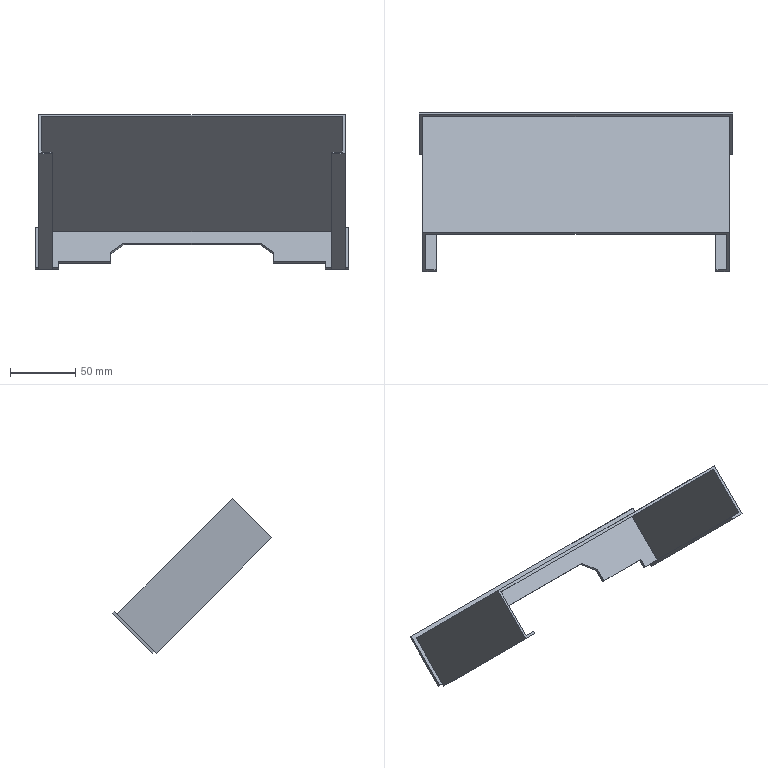Component | SolidWorks | Section4-1 | 2 solids | 30 faces | box 240 x 121.98 x 118.44 mm | volume 96218 mm3 | plane 30
build123d program:
from build123d import *

# Parameters (mm, degrees)
EXTRUDE_THIN1_DEPTH = 125
BOSS_EXTRUDE1_DEPTH = 2


with BuildPart() as part:
    # Sketch1 → Extrude-Thin1 (new body)
    with BuildSketch(Plane.XY):
        Polygon((2151.948, -29.605), (2141.948, -29.605), (2141.948, 12.895), (2375.948, 12.895), (2375.948, -29.605), (2365.948, -29.605), (2365.948, -27.605), (2373.948, -27.605), (2373.948, 10.895), (2143.948, 10.895), (2143.948, -27.605), (2151.948, -27.605), align=None)
    extrude(amount=EXTRUDE_THIN1_DEPTH)


with BuildPart() as body_2:
    # Sketch2 → Boss-Extrude1 (new body)
    with BuildSketch(Plane(origin=(0, 0, 0), x_dir=(-1, 0, 0), z_dir=(0, 0, -1))):
        Polygon((-2360.948, -27.605), (-2378.948, -27.605), (-2378.948, 15.895), (-2138.948, 15.895), (-2138.948, -27.605), (-2156.948, -27.605), (-2156.948, -21.105), (-2196.948, -21.105), (-2196.948, -11.105), (-2206.948, -1.105), (-2310.948, -1.105), (-2320.948, -11.105), (-2320.948, -21.105), (-2360.948, -21.105), align=None)
    extrude(amount=BOSS_EXTRUDE1_DEPTH)


solid = Compound([part.part, body_2.part])

# Placed as in the assembly
solid = solid.moved(Location((-2140.123, -346.52, 136.747), (45, 0, 0)))
STEP:
#1=COLOUR_RGB('',0.7922,0.8196,0.9333);
#2=FILL_AREA_STYLE_COLOUR('',#1);
#3=FILL_AREA_STYLE('',(#2));
#4=SURFACE_STYLE_FILL_AREA(#3);
#5=SURFACE_SIDE_STYLE('',(#4));
#6=SURFACE_STYLE_USAGE(.BOTH.,#5);
#7=PRESENTATION_STYLE_ASSIGNMENT((#6));
#8=CARTESIAN_POINT('',(8.694,-14.411,4.615));
#9=VERTEX_POINT('',#8);
#10=CARTESIAN_POINT('',(8.694,-14.23,4.796));
#11=VERTEX_POINT('',#10);
#12=CARTESIAN_POINT('',(8.694,-14.23,4.796));
#13=DIRECTION('',(-0.,0.7071,0.7071));
#14=VECTOR('',#13,39.37);
#15=LINE('',#12,#14);
#16=EDGE_CURVE('',#9,#11,#15,.T.);
#17=ORIENTED_EDGE('',*,*,#16,.T.);
#18=CARTESIAN_POINT('',(8.694,-14.174,4.741));
#19=VERTEX_POINT('',#18);
#20=CARTESIAN_POINT('',(8.694,-14.174,4.741));
#21=DIRECTION('',(0.,-0.7071,0.7071));
#22=VECTOR('',#21,39.37);
#23=LINE('',#20,#22);
#24=EDGE_CURVE('',#19,#11,#23,.T.);
#25=ORIENTED_EDGE('',*,*,#24,.F.);
#26=CARTESIAN_POINT('',(8.694,-14.355,4.56));
#27=VERTEX_POINT('',#26);
#28=CARTESIAN_POINT('',(8.694,-14.174,4.741));
#29=DIRECTION('',(-0.,0.7071,0.7071));
#30=VECTOR('',#29,39.37);
#31=LINE('',#28,#30);
#32=EDGE_CURVE('',#27,#19,#31,.T.);
#33=ORIENTED_EDGE('',*,*,#32,.F.);
#34=CARTESIAN_POINT('',(8.694,-14.355,4.56));
#35=DIRECTION('',(0.,-0.7071,0.7071));
#36=VECTOR('',#35,39.37);
#37=LINE('',#34,#36);
#38=EDGE_CURVE('',#27,#9,#37,.T.);
#39=ORIENTED_EDGE('',*,*,#38,.T.);
#40=EDGE_LOOP('',(#17,#25,#33,#39));
#41=FACE_OUTER_BOUND('',#40,.T.);
#42=CARTESIAN_POINT('',(8.694,-14.174,4.741));
#43=DIRECTION('',(1.,0.,-0.));
#44=DIRECTION('',(-0.,0.7071,-0.7071));
#45=AXIS2_PLACEMENT_3D('',#42,#43,#44);
#46=PLANE('',#45);
#47=ADVANCED_FACE('',(#41),#46,.F.);
#48=CARTESIAN_POINT('',(7.119,-14.23,4.796));
#49=VERTEX_POINT('',#48);
#50=CARTESIAN_POINT('',(7.119,-14.23,4.796));
#51=DIRECTION('',(-1.,-0.,0.));
#52=VECTOR('',#51,39.37);
#53=LINE('',#50,#52);
#54=EDGE_CURVE('',#11,#49,#53,.T.);
#55=ORIENTED_EDGE('',*,*,#54,.T.);
#56=CARTESIAN_POINT('',(7.119,-14.174,4.741));
#57=VERTEX_POINT('',#56);
#58=CARTESIAN_POINT('',(7.119,-14.174,4.741));
#59=DIRECTION('',(0.,-0.7071,0.7071));
#60=VECTOR('',#59,39.37);
#61=LINE('',#58,#60);
#62=EDGE_CURVE('',#57,#49,#61,.T.);
#63=ORIENTED_EDGE('',*,*,#62,.F.);
#64=CARTESIAN_POINT('',(7.119,-14.174,4.741));
#65=DIRECTION('',(-1.,-0.,0.));
#66=VECTOR('',#65,39.37);
#67=LINE('',#64,#66);
#68=EDGE_CURVE('',#19,#57,#67,.T.);
#69=ORIENTED_EDGE('',*,*,#68,.F.);
#70=ORIENTED_EDGE('',*,*,#24,.T.);
#71=EDGE_LOOP('',(#55,#63,#69,#70));
#72=FACE_OUTER_BOUND('',#71,.T.);
#73=CARTESIAN_POINT('',(7.119,-14.174,4.741));
#74=DIRECTION('',(0.,0.7071,0.7071));
#75=DIRECTION('',(-1.,-0.,0.));
#76=AXIS2_PLACEMENT_3D('',#73,#74,#75);
#77=PLANE('',#76);
#78=ADVANCED_FACE('',(#72),#77,.F.);
#79=CARTESIAN_POINT('',(7.119,-13.952,5.075));
#80=VERTEX_POINT('',#79);
#81=CARTESIAN_POINT('',(7.119,-13.952,5.075));
#82=DIRECTION('',(0.,0.7071,0.7071));
#83=VECTOR('',#82,39.37);
#84=LINE('',#81,#83);
#85=EDGE_CURVE('',#49,#80,#84,.T.);
#86=ORIENTED_EDGE('',*,*,#85,.T.);
#87=CARTESIAN_POINT('',(7.119,-13.896,5.019));
#88=VERTEX_POINT('',#87);
#89=CARTESIAN_POINT('',(7.119,-13.896,5.019));
#90=DIRECTION('',(0.,-0.7071,0.7071));
#91=VECTOR('',#90,39.37);
#92=LINE('',#89,#91);
#93=EDGE_CURVE('',#88,#80,#92,.T.);
#94=ORIENTED_EDGE('',*,*,#93,.F.);
#95=CARTESIAN_POINT('',(7.119,-13.896,5.019));
#96=DIRECTION('',(0.,0.7071,0.7071));
#97=VECTOR('',#96,39.37);
#98=LINE('',#95,#97);
#99=EDGE_CURVE('',#57,#88,#98,.T.);
#100=ORIENTED_EDGE('',*,*,#99,.F.);
#101=ORIENTED_EDGE('',*,*,#62,.T.);
#102=EDGE_LOOP('',(#86,#94,#100,#101));
#103=FACE_OUTER_BOUND('',#102,.T.);
#104=CARTESIAN_POINT('',(7.119,-13.896,5.019));
#105=DIRECTION('',(1.,-0.,-0.));
#106=DIRECTION('',(0.,0.7071,0.7071));
#107=AXIS2_PLACEMENT_3D('',#104,#105,#106);
#108=PLANE('',#107);
#109=ADVANCED_FACE('',(#103),#108,.F.);
#110=CARTESIAN_POINT('',(6.725,-13.673,5.353));
#111=VERTEX_POINT('',#110);
#112=CARTESIAN_POINT('',(6.725,-13.673,5.353));
#113=DIRECTION('',(-0.7071,0.5,0.5));
#114=VECTOR('',#113,39.37);
#115=LINE('',#112,#114);
#116=EDGE_CURVE('',#80,#111,#115,.T.);
#117=ORIENTED_EDGE('',*,*,#116,.T.);
#118=CARTESIAN_POINT('',(6.725,-13.618,5.297));
#119=VERTEX_POINT('',#118);
#120=CARTESIAN_POINT('',(6.725,-13.618,5.297));
#121=DIRECTION('',(0.,-0.7071,0.7071));
#122=VECTOR('',#121,39.37);
#123=LINE('',#120,#122);
#124=EDGE_CURVE('',#119,#111,#123,.T.);
#125=ORIENTED_EDGE('',*,*,#124,.F.);
#126=CARTESIAN_POINT('',(6.725,-13.618,5.297));
#127=DIRECTION('',(-0.7071,0.5,0.5));
#128=VECTOR('',#127,39.37);
#129=LINE('',#126,#128);
#130=EDGE_CURVE('',#88,#119,#129,.T.);
#131=ORIENTED_EDGE('',*,*,#130,.F.);
#132=ORIENTED_EDGE('',*,*,#93,.T.);
#133=EDGE_LOOP('',(#117,#125,#131,#132));
#134=FACE_OUTER_BOUND('',#133,.T.);
#135=CARTESIAN_POINT('',(6.725,-13.618,5.297));
#136=DIRECTION('',(0.7071,0.5,0.5));
#137=DIRECTION('',(-0.7071,0.5,0.5));
#138=AXIS2_PLACEMENT_3D('',#135,#136,#137);
#139=PLANE('',#138);
#140=ADVANCED_FACE('',(#134),#139,.F.);
#141=CARTESIAN_POINT('',(2.631,-13.673,5.353));
#142=VERTEX_POINT('',#141);
#143=CARTESIAN_POINT('',(2.631,-13.673,5.353));
#144=DIRECTION('',(-1.,-0.,0.));
#145=VECTOR('',#144,39.37);
#146=LINE('',#143,#145);
#147=EDGE_CURVE('',#111,#142,#146,.T.);
#148=ORIENTED_EDGE('',*,*,#147,.T.);
#149=CARTESIAN_POINT('',(2.631,-13.618,5.297));
#150=VERTEX_POINT('',#149);
#151=CARTESIAN_POINT('',(2.631,-13.618,5.297));
#152=DIRECTION('',(0.,-0.7071,0.7071));
#153=VECTOR('',#152,39.37);
#154=LINE('',#151,#153);
#155=EDGE_CURVE('',#150,#142,#154,.T.);
#156=ORIENTED_EDGE('',*,*,#155,.F.);
#157=CARTESIAN_POINT('',(2.631,-13.618,5.297));
#158=DIRECTION('',(-1.,-0.,0.));
#159=VECTOR('',#158,39.37);
#160=LINE('',#157,#159);
#161=EDGE_CURVE('',#119,#150,#160,.T.);
#162=ORIENTED_EDGE('',*,*,#161,.F.);
#163=ORIENTED_EDGE('',*,*,#124,.T.);
#164=EDGE_LOOP('',(#148,#156,#162,#163));
#165=FACE_OUTER_BOUND('',#164,.T.);
#166=CARTESIAN_POINT('',(2.631,-13.618,5.297));
#167=DIRECTION('',(0.,0.7071,0.7071));
#168=DIRECTION('',(-1.,-0.,0.));
#169=AXIS2_PLACEMENT_3D('',#166,#167,#168);
#170=PLANE('',#169);
#171=ADVANCED_FACE('',(#165),#170,.F.);
#172=CARTESIAN_POINT('',(2.237,-13.952,5.075));
#173=VERTEX_POINT('',#172);
#174=CARTESIAN_POINT('',(2.237,-13.952,5.075));
#175=DIRECTION('',(-0.7071,-0.5,-0.5));
#176=VECTOR('',#175,39.37);
#177=LINE('',#174,#176);
#178=EDGE_CURVE('',#142,#173,#177,.T.);
#179=ORIENTED_EDGE('',*,*,#178,.T.);
#180=CARTESIAN_POINT('',(2.237,-13.896,5.019));
#181=VERTEX_POINT('',#180);
#182=CARTESIAN_POINT('',(2.237,-13.896,5.019));
#183=DIRECTION('',(0.,-0.7071,0.7071));
#184=VECTOR('',#183,39.37);
#185=LINE('',#182,#184);
#186=EDGE_CURVE('',#181,#173,#185,.T.);
#187=ORIENTED_EDGE('',*,*,#186,.F.);
#188=CARTESIAN_POINT('',(2.237,-13.896,5.019));
#189=DIRECTION('',(-0.7071,-0.5,-0.5));
#190=VECTOR('',#189,39.37);
#191=LINE('',#188,#190);
#192=EDGE_CURVE('',#150,#181,#191,.T.);
#193=ORIENTED_EDGE('',*,*,#192,.F.);
#194=ORIENTED_EDGE('',*,*,#155,.T.);
#195=EDGE_LOOP('',(#179,#187,#193,#194));
#196=FACE_OUTER_BOUND('',#195,.T.);
#197=CARTESIAN_POINT('',(2.237,-13.896,5.019));
#198=DIRECTION('',(-0.7071,0.5,0.5));
#199=DIRECTION('',(-0.7071,-0.5,-0.5));
#200=AXIS2_PLACEMENT_3D('',#197,#198,#199);
#201=PLANE('',#200);
#202=ADVANCED_FACE('',(#196),#201,.F.);
#203=CARTESIAN_POINT('',(2.237,-14.23,4.796));
#204=VERTEX_POINT('',#203);
#205=CARTESIAN_POINT('',(2.237,-14.23,4.796));
#206=DIRECTION('',(-0.,-0.7071,-0.7071));
#207=VECTOR('',#206,39.37);
#208=LINE('',#205,#207);
#209=EDGE_CURVE('',#173,#204,#208,.T.);
#210=ORIENTED_EDGE('',*,*,#209,.T.);
#211=CARTESIAN_POINT('',(2.237,-14.174,4.741));
#212=VERTEX_POINT('',#211);
#213=CARTESIAN_POINT('',(2.237,-14.174,4.741));
#214=DIRECTION('',(0.,-0.7071,0.7071));
#215=VECTOR('',#214,39.37);
#216=LINE('',#213,#215);
#217=EDGE_CURVE('',#212,#204,#216,.T.);
#218=ORIENTED_EDGE('',*,*,#217,.F.);
#219=CARTESIAN_POINT('',(2.237,-14.174,4.741));
#220=DIRECTION('',(-0.,-0.7071,-0.7071));
#221=VECTOR('',#220,39.37);
#222=LINE('',#219,#221);
#223=EDGE_CURVE('',#181,#212,#222,.T.);
#224=ORIENTED_EDGE('',*,*,#223,.F.);
#225=ORIENTED_EDGE('',*,*,#186,.T.);
#226=EDGE_LOOP('',(#210,#218,#224,#225));
#227=FACE_OUTER_BOUND('',#226,.T.);
#228=CARTESIAN_POINT('',(2.237,-14.174,4.741));
#229=DIRECTION('',(-1.,0.,0.));
#230=DIRECTION('',(-0.,-0.7071,-0.7071));
#231=AXIS2_PLACEMENT_3D('',#228,#229,#230);
#232=PLANE('',#231);
#233=ADVANCED_FACE('',(#227),#232,.F.);
#234=CARTESIAN_POINT('',(0.6624,-14.23,4.796));
#235=VERTEX_POINT('',#234);
#236=CARTESIAN_POINT('',(0.6624,-14.23,4.796));
#237=DIRECTION('',(-1.,-0.,0.));
#238=VECTOR('',#237,39.37);
#239=LINE('',#236,#238);
#240=EDGE_CURVE('',#204,#235,#239,.T.);
#241=ORIENTED_EDGE('',*,*,#240,.T.);
#242=CARTESIAN_POINT('',(0.6624,-14.174,4.741));
#243=VERTEX_POINT('',#242);
#244=CARTESIAN_POINT('',(0.6624,-14.174,4.741));
#245=DIRECTION('',(0.,-0.7071,0.7071));
#246=VECTOR('',#245,39.37);
#247=LINE('',#244,#246);
#248=EDGE_CURVE('',#243,#235,#247,.T.);
#249=ORIENTED_EDGE('',*,*,#248,.F.);
#250=CARTESIAN_POINT('',(0.6624,-14.174,4.741));
#251=DIRECTION('',(-1.,-0.,0.));
#252=VECTOR('',#251,39.37);
#253=LINE('',#250,#252);
#254=EDGE_CURVE('',#212,#243,#253,.T.);
#255=ORIENTED_EDGE('',*,*,#254,.F.);
#256=ORIENTED_EDGE('',*,*,#217,.T.);
#257=EDGE_LOOP('',(#241,#249,#255,#256));
#258=FACE_OUTER_BOUND('',#257,.T.);
#259=CARTESIAN_POINT('',(0.6624,-14.174,4.741));
#260=DIRECTION('',(0.,0.7071,0.7071));
#261=DIRECTION('',(-1.,-0.,0.));
#262=AXIS2_PLACEMENT_3D('',#259,#260,#261);
#263=PLANE('',#262);
#264=ADVANCED_FACE('',(#258),#263,.F.);
#265=CARTESIAN_POINT('',(0.6624,-14.411,4.615));
#266=VERTEX_POINT('',#265);
#267=CARTESIAN_POINT('',(0.6624,-14.411,4.615));
#268=DIRECTION('',(0.,-0.7071,-0.7071));
#269=VECTOR('',#268,39.37);
#270=LINE('',#267,#269);
#271=EDGE_CURVE('',#235,#266,#270,.T.);
#272=ORIENTED_EDGE('',*,*,#271,.T.);
#273=CARTESIAN_POINT('',(0.6624,-14.355,4.56));
#274=VERTEX_POINT('',#273);
#275=CARTESIAN_POINT('',(0.6624,-14.355,4.56));
#276=DIRECTION('',(0.,-0.7071,0.7071));
#277=VECTOR('',#276,39.37);
#278=LINE('',#275,#277);
#279=EDGE_CURVE('',#274,#266,#278,.T.);
#280=ORIENTED_EDGE('',*,*,#279,.F.);
#281=CARTESIAN_POINT('',(0.6624,-14.355,4.56));
#282=DIRECTION('',(0.,-0.7071,-0.7071));
#283=VECTOR('',#282,39.37);
#284=LINE('',#281,#283);
#285=EDGE_CURVE('',#243,#274,#284,.T.);
#286=ORIENTED_EDGE('',*,*,#285,.F.);
#287=ORIENTED_EDGE('',*,*,#248,.T.);
#288=EDGE_LOOP('',(#272,#280,#286,#287));
#289=FACE_OUTER_BOUND('',#288,.T.);
#290=CARTESIAN_POINT('',(0.6624,-14.355,4.56));
#291=DIRECTION('',(-1.,-0.,0.));
#292=DIRECTION('',(0.,-0.7071,0.7071));
#293=AXIS2_PLACEMENT_3D('',#290,#291,#292);
#294=PLANE('',#293);
#295=ADVANCED_FACE('',(#289),#294,.F.);
#296=CARTESIAN_POINT('',(-0.04628,-14.411,4.615));
#297=VERTEX_POINT('',#296);
#298=CARTESIAN_POINT('',(-0.04628,-14.411,4.615));
#299=DIRECTION('',(-1.,-0.,0.));
#300=VECTOR('',#299,39.37);
#301=LINE('',#298,#300);
#302=EDGE_CURVE('',#266,#297,#301,.T.);
#303=ORIENTED_EDGE('',*,*,#302,.T.);
#304=CARTESIAN_POINT('',(-0.04628,-14.355,4.56));
#305=VERTEX_POINT('',#304);
#306=CARTESIAN_POINT('',(-0.04628,-14.355,4.56));
#307=DIRECTION('',(0.,-0.7071,0.7071));
#308=VECTOR('',#307,39.37);
#309=LINE('',#306,#308);
#310=EDGE_CURVE('',#305,#297,#309,.T.);
#311=ORIENTED_EDGE('',*,*,#310,.F.);
#312=CARTESIAN_POINT('',(-0.04628,-14.355,4.56));
#313=DIRECTION('',(-1.,-0.,0.));
#314=VECTOR('',#313,39.37);
#315=LINE('',#312,#314);
#316=EDGE_CURVE('',#274,#305,#315,.T.);
#317=ORIENTED_EDGE('',*,*,#316,.F.);
#318=ORIENTED_EDGE('',*,*,#279,.T.);
#319=EDGE_LOOP('',(#303,#311,#317,#318));
#320=FACE_OUTER_BOUND('',#319,.T.);
#321=CARTESIAN_POINT('',(-0.04628,-14.355,4.56));
#322=DIRECTION('',(-0.,0.7071,0.7071));
#323=DIRECTION('',(0.,-0.7071,0.7071));
#324=AXIS2_PLACEMENT_3D('',#321,#322,#323);
#325=PLANE('',#324);
#326=ADVANCED_FACE('',(#320),#325,.F.);
#327=CARTESIAN_POINT('',(-0.04628,-13.2,5.826));
#328=VERTEX_POINT('',#327);
#329=CARTESIAN_POINT('',(-0.04628,-13.2,5.826));
#330=DIRECTION('',(-0.,0.7071,0.7071));
#331=VECTOR('',#330,39.37);
#332=LINE('',#329,#331);
#333=EDGE_CURVE('',#297,#328,#332,.T.);
#334=ORIENTED_EDGE('',*,*,#333,.T.);
#335=CARTESIAN_POINT('',(-0.04628,-13.144,5.771));
#336=VERTEX_POINT('',#335);
#337=CARTESIAN_POINT('',(-0.04628,-13.144,5.771));
#338=DIRECTION('',(0.,-0.7071,0.7071));
#339=VECTOR('',#338,39.37);
#340=LINE('',#337,#339);
#341=EDGE_CURVE('',#336,#328,#340,.T.);
#342=ORIENTED_EDGE('',*,*,#341,.F.);
#343=CARTESIAN_POINT('',(-0.04628,-13.144,5.771));
#344=DIRECTION('',(-0.,0.7071,0.7071));
#345=VECTOR('',#344,39.37);
#346=LINE('',#343,#345);
#347=EDGE_CURVE('',#305,#336,#346,.T.);
#348=ORIENTED_EDGE('',*,*,#347,.F.);
#349=ORIENTED_EDGE('',*,*,#310,.T.);
#350=EDGE_LOOP('',(#334,#342,#348,#349));
#351=FACE_OUTER_BOUND('',#350,.T.);
#352=CARTESIAN_POINT('',(-0.04628,-13.144,5.771));
#353=DIRECTION('',(1.,0.,-0.));
#354=DIRECTION('',(-0.,0.7071,-0.7071));
#355=AXIS2_PLACEMENT_3D('',#352,#353,#354);
#356=PLANE('',#355);
#357=ADVANCED_FACE('',(#351),#356,.F.);
#358=CARTESIAN_POINT('',(9.403,-13.2,5.826));
#359=VERTEX_POINT('',#358);
#360=CARTESIAN_POINT('',(9.403,-13.2,5.826));
#361=DIRECTION('',(1.,0.,-0.));
#362=VECTOR('',#361,39.37);
#363=LINE('',#360,#362);
#364=EDGE_CURVE('',#328,#359,#363,.T.);
#365=ORIENTED_EDGE('',*,*,#364,.T.);
#366=CARTESIAN_POINT('',(9.403,-13.144,5.771));
#367=VERTEX_POINT('',#366);
#368=CARTESIAN_POINT('',(9.403,-13.144,5.771));
#369=DIRECTION('',(0.,-0.7071,0.7071));
#370=VECTOR('',#369,39.37);
#371=LINE('',#368,#370);
#372=EDGE_CURVE('',#367,#359,#371,.T.);
#373=ORIENTED_EDGE('',*,*,#372,.F.);
#374=CARTESIAN_POINT('',(9.403,-13.144,5.771));
#375=DIRECTION('',(1.,0.,-0.));
#376=VECTOR('',#375,39.37);
#377=LINE('',#374,#376);
#378=EDGE_CURVE('',#336,#367,#377,.T.);
#379=ORIENTED_EDGE('',*,*,#378,.F.);
#380=ORIENTED_EDGE('',*,*,#341,.T.);
#381=EDGE_LOOP('',(#365,#373,#379,#380));
#382=FACE_OUTER_BOUND('',#381,.T.);
#383=CARTESIAN_POINT('',(9.403,-13.144,5.771));
#384=DIRECTION('',(0.,-0.7071,-0.7071));
#385=DIRECTION('',(-0.,0.7071,-0.7071));
#386=AXIS2_PLACEMENT_3D('',#383,#384,#385);
#387=PLANE('',#386);
#388=ADVANCED_FACE('',(#382),#387,.F.);
#389=CARTESIAN_POINT('',(9.403,-14.411,4.615));
#390=VERTEX_POINT('',#389);
#391=CARTESIAN_POINT('',(9.403,-14.411,4.615));
#392=DIRECTION('',(0.,-0.7071,-0.7071));
#393=VECTOR('',#392,39.37);
#394=LINE('',#391,#393);
#395=EDGE_CURVE('',#359,#390,#394,.T.);
#396=ORIENTED_EDGE('',*,*,#395,.T.);
#397=CARTESIAN_POINT('',(9.403,-14.355,4.56));
#398=VERTEX_POINT('',#397);
#399=CARTESIAN_POINT('',(9.403,-14.355,4.56));
#400=DIRECTION('',(0.,-0.7071,0.7071));
#401=VECTOR('',#400,39.37);
#402=LINE('',#399,#401);
#403=EDGE_CURVE('',#398,#390,#402,.T.);
#404=ORIENTED_EDGE('',*,*,#403,.F.);
#405=CARTESIAN_POINT('',(9.403,-14.355,4.56));
#406=DIRECTION('',(0.,-0.7071,-0.7071));
#407=VECTOR('',#406,39.37);
#408=LINE('',#405,#407);
#409=EDGE_CURVE('',#367,#398,#408,.T.);
#410=ORIENTED_EDGE('',*,*,#409,.F.);
#411=ORIENTED_EDGE('',*,*,#372,.T.);
#412=EDGE_LOOP('',(#396,#404,#410,#411));
#413=FACE_OUTER_BOUND('',#412,.T.);
#414=CARTESIAN_POINT('',(9.403,-14.355,4.56));
#415=DIRECTION('',(-1.,-0.,0.));
#416=DIRECTION('',(0.,-0.7071,0.7071));
#417=AXIS2_PLACEMENT_3D('',#414,#415,#416);
#418=PLANE('',#417);
#419=ADVANCED_FACE('',(#413),#418,.F.);
#420=CARTESIAN_POINT('',(8.694,-14.411,4.615));
#421=DIRECTION('',(-1.,-0.,0.));
#422=VECTOR('',#421,39.37);
#423=LINE('',#420,#422);
#424=EDGE_CURVE('',#390,#9,#423,.T.);
#425=ORIENTED_EDGE('',*,*,#424,.T.);
#426=ORIENTED_EDGE('',*,*,#38,.F.);
#427=CARTESIAN_POINT('',(8.694,-14.355,4.56));
#428=DIRECTION('',(-1.,-0.,0.));
#429=VECTOR('',#428,39.37);
#430=LINE('',#427,#429);
#431=EDGE_CURVE('',#398,#27,#430,.T.);
#432=ORIENTED_EDGE('',*,*,#431,.F.);
#433=ORIENTED_EDGE('',*,*,#403,.T.);
#434=EDGE_LOOP('',(#425,#426,#432,#433));
#435=FACE_OUTER_BOUND('',#434,.T.);
#436=CARTESIAN_POINT('',(8.694,-14.355,4.56));
#437=DIRECTION('',(-0.,0.7071,0.7071));
#438=DIRECTION('',(0.,-0.7071,0.7071));
#439=AXIS2_PLACEMENT_3D('',#436,#437,#438);
#440=PLANE('',#439);
#441=ADVANCED_FACE('',(#435),#440,.F.);
#442=ORIENTED_EDGE('',*,*,#32,.T.);
#443=ORIENTED_EDGE('',*,*,#68,.T.);
#444=ORIENTED_EDGE('',*,*,#99,.T.);
#445=ORIENTED_EDGE('',*,*,#130,.T.);
#446=ORIENTED_EDGE('',*,*,#161,.T.);
#447=ORIENTED_EDGE('',*,*,#192,.T.);
#448=ORIENTED_EDGE('',*,*,#223,.T.);
#449=ORIENTED_EDGE('',*,*,#254,.T.);
#450=ORIENTED_EDGE('',*,*,#285,.T.);
#451=ORIENTED_EDGE('',*,*,#316,.T.);
#452=ORIENTED_EDGE('',*,*,#347,.T.);
#453=ORIENTED_EDGE('',*,*,#378,.T.);
#454=ORIENTED_EDGE('',*,*,#409,.T.);
#455=ORIENTED_EDGE('',*,*,#431,.T.);
#456=EDGE_LOOP('',(#442,#443,#444,#445,#446,#447,#448,#449,#450,#451,#452,#453,#454,#455));
#457=FACE_OUTER_BOUND('',#456,.T.);
#458=CARTESIAN_POINT('',(-84.257,-13.587,5.328));
#459=DIRECTION('',(0.,-0.7071,0.7071));
#460=DIRECTION('',(1.,0.,-0.));
#461=AXIS2_PLACEMENT_3D('',#458,#459,#460);
#462=PLANE('',#461);
#463=ADVANCED_FACE('',(#457),#462,.F.);
#464=ORIENTED_EDGE('',*,*,#16,.F.);
#465=ORIENTED_EDGE('',*,*,#424,.F.);
#466=ORIENTED_EDGE('',*,*,#395,.F.);
#467=ORIENTED_EDGE('',*,*,#364,.F.);
#468=ORIENTED_EDGE('',*,*,#333,.F.);
#469=ORIENTED_EDGE('',*,*,#302,.F.);
#470=ORIENTED_EDGE('',*,*,#271,.F.);
#471=ORIENTED_EDGE('',*,*,#240,.F.);
#472=ORIENTED_EDGE('',*,*,#209,.F.);
#473=ORIENTED_EDGE('',*,*,#178,.F.);
#474=ORIENTED_EDGE('',*,*,#147,.F.);
#475=ORIENTED_EDGE('',*,*,#116,.F.);
#476=ORIENTED_EDGE('',*,*,#85,.F.);
#477=ORIENTED_EDGE('',*,*,#54,.F.);
#478=EDGE_LOOP('',(#464,#465,#466,#467,#468,#469,#470,#471,#472,#473,#474,#475,#476,#477));
#479=FACE_OUTER_BOUND('',#478,.T.);
#480=CARTESIAN_POINT('',(-84.257,-13.643,5.384));
#481=DIRECTION('',(0.,-0.7071,0.7071));
#482=DIRECTION('',(1.,0.,-0.));
#483=AXIS2_PLACEMENT_3D('',#480,#481,#482);
#484=PLANE('',#483);
#485=ADVANCED_FACE('',(#479),#484,.T.);
#486=CLOSED_SHELL('',(#47,#78,#109,#140,#171,#202,#233,#264,#295,#326,#357,#388,#419,#441,#463,#485));
#487=MANIFOLD_SOLID_BREP('',#486);
#488=STYLED_ITEM('',(#7),#487);
#489=(LENGTH_UNIT()NAMED_UNIT(*)SI_UNIT($,.METRE.));
#490=LENGTH_MEASURE_WITH_UNIT(LENGTH_MEASURE(0.0254),#489);
#491=DIMENSIONAL_EXPONENTS(1.,0.,0.,0.,0.,0.,0.);
#492=(CONVERSION_BASED_UNIT('',#490)LENGTH_UNIT()NAMED_UNIT(#491));
#493=UNCERTAINTY_MEASURE_WITH_UNIT(LENGTH_MEASURE(0.00001),#492,'','');
#494=(NAMED_UNIT(*)PLANE_ANGLE_UNIT()SI_UNIT($,.RADIAN.));
#495=(NAMED_UNIT(*)SI_UNIT($,.STERADIAN.)SOLID_ANGLE_UNIT());
#496=(GEOMETRIC_REPRESENTATION_CONTEXT(3)GLOBAL_UNCERTAINTY_ASSIGNED_CONTEXT((#493))GLOBAL_UNIT_ASSIGNED_CONTEXT((#492,#494,#495))REPRESENTATION_CONTEXT('',''));
#497=MECHANICAL_DESIGN_GEOMETRIC_PRESENTATION_REPRESENTATION('',(#488),#496);
#498=COLOUR_RGB('',0.7922,0.8196,0.9333);
#499=FILL_AREA_STYLE_COLOUR('',#498);
#500=FILL_AREA_STYLE('',(#499));
#501=SURFACE_STYLE_FILL_AREA(#500);
#502=SURFACE_SIDE_STYLE('',(#501));
#503=SURFACE_STYLE_USAGE(.BOTH.,#502);
#504=PRESENTATION_STYLE_ASSIGNMENT((#503));
#505=CARTESIAN_POINT('',(0.07183,-14.467,4.56));
#506=VERTEX_POINT('',#505);
#507=CARTESIAN_POINT('',(0.4655,-14.467,4.56));
#508=VERTEX_POINT('',#507);
#509=CARTESIAN_POINT('',(0.07183,-14.467,4.56));
#510=DIRECTION('',(1.,0.,-0.));
#511=VECTOR('',#510,39.37);
#512=LINE('',#509,#511);
#513=EDGE_CURVE('',#506,#508,#512,.T.);
#514=ORIENTED_EDGE('',*,*,#513,.T.);
#515=CARTESIAN_POINT('',(0.4655,-17.947,8.039));
#516=VERTEX_POINT('',#515);
#517=CARTESIAN_POINT('',(0.4655,-17.947,8.039));
#518=DIRECTION('',(-0.,0.7071,-0.7071));
#519=VECTOR('',#518,39.37);
#520=LINE('',#517,#519);
#521=EDGE_CURVE('',#516,#508,#520,.T.);
#522=ORIENTED_EDGE('',*,*,#521,.F.);
#523=CARTESIAN_POINT('',(0.07183,-17.947,8.039));
#524=VERTEX_POINT('',#523);
#525=CARTESIAN_POINT('',(0.07183,-17.947,8.039));
#526=DIRECTION('',(1.,0.,-0.));
#527=VECTOR('',#526,39.37);
#528=LINE('',#525,#527);
#529=EDGE_CURVE('',#524,#516,#528,.T.);
#530=ORIENTED_EDGE('',*,*,#529,.F.);
#531=CARTESIAN_POINT('',(0.07183,-17.947,8.039));
#532=DIRECTION('',(-0.,0.7071,-0.7071));
#533=VECTOR('',#532,39.37);
#534=LINE('',#531,#533);
#535=EDGE_CURVE('',#524,#506,#534,.T.);
#536=ORIENTED_EDGE('',*,*,#535,.T.);
#537=EDGE_LOOP('',(#514,#522,#530,#536));
#538=FACE_OUTER_BOUND('',#537,.T.);
#539=CARTESIAN_POINT('',(0.07183,-17.947,8.039));
#540=DIRECTION('',(-0.,0.7071,0.7071));
#541=DIRECTION('',(0.,-0.7071,0.7071));
#542=AXIS2_PLACEMENT_3D('',#539,#540,#541);
#543=PLANE('',#542);
#544=ADVANCED_FACE('',(#538),#543,.F.);
#545=CARTESIAN_POINT('',(0.4655,-14.411,4.615));
#546=VERTEX_POINT('',#545);
#547=CARTESIAN_POINT('',(0.4655,-14.411,4.615));
#548=DIRECTION('',(0.,-0.7071,-0.7071));
#549=VECTOR('',#548,39.37);
#550=LINE('',#547,#549);
#551=EDGE_CURVE('',#546,#508,#550,.T.);
#552=ORIENTED_EDGE('',*,*,#551,.F.);
#553=CARTESIAN_POINT('',(0.4655,-17.891,8.095));
#554=VERTEX_POINT('',#553);
#555=CARTESIAN_POINT('',(0.4655,-17.891,8.095));
#556=DIRECTION('',(-0.,0.7071,-0.7071));
#557=VECTOR('',#556,39.37);
#558=LINE('',#555,#557);
#559=EDGE_CURVE('',#554,#546,#558,.T.);
#560=ORIENTED_EDGE('',*,*,#559,.F.);
#561=CARTESIAN_POINT('',(0.4655,-17.891,8.095));
#562=DIRECTION('',(0.,-0.7071,-0.7071));
#563=VECTOR('',#562,39.37);
#564=LINE('',#561,#563);
#565=EDGE_CURVE('',#554,#516,#564,.T.);
#566=ORIENTED_EDGE('',*,*,#565,.T.);
#567=ORIENTED_EDGE('',*,*,#521,.T.);
#568=EDGE_LOOP('',(#552,#560,#566,#567));
#569=FACE_OUTER_BOUND('',#568,.T.);
#570=CARTESIAN_POINT('',(0.4655,-17.891,8.095));
#571=DIRECTION('',(1.,0.,-0.));
#572=DIRECTION('',(-0.,0.7071,-0.7071));
#573=AXIS2_PLACEMENT_3D('',#570,#571,#572);
#574=PLANE('',#573);
#575=ADVANCED_FACE('',(#569),#574,.T.);
#576=CARTESIAN_POINT('',(0.1506,-14.411,4.615));
#577=VERTEX_POINT('',#576);
#578=CARTESIAN_POINT('',(0.07183,-14.411,4.615));
#579=DIRECTION('',(1.,0.,-0.));
#580=VECTOR('',#579,39.37);
#581=LINE('',#578,#580);
#582=EDGE_CURVE('',#577,#546,#581,.T.);
#583=ORIENTED_EDGE('',*,*,#582,.F.);
#584=CARTESIAN_POINT('',(0.1506,-17.891,8.095));
#585=VERTEX_POINT('',#584);
#586=CARTESIAN_POINT('',(0.1506,-17.891,8.095));
#587=DIRECTION('',(-0.,0.7071,-0.7071));
#588=VECTOR('',#587,39.37);
#589=LINE('',#586,#588);
#590=EDGE_CURVE('',#585,#577,#589,.T.);
#591=ORIENTED_EDGE('',*,*,#590,.F.);
#592=CARTESIAN_POINT('',(0.07183,-17.891,8.095));
#593=DIRECTION('',(1.,0.,-0.));
#594=VECTOR('',#593,39.37);
#595=LINE('',#592,#594);
#596=EDGE_CURVE('',#585,#554,#595,.T.);
#597=ORIENTED_EDGE('',*,*,#596,.T.);
#598=ORIENTED_EDGE('',*,*,#559,.T.);
#599=EDGE_LOOP('',(#583,#591,#597,#598));
#600=FACE_OUTER_BOUND('',#599,.T.);
#601=CARTESIAN_POINT('',(0.07183,-17.891,8.095));
#602=DIRECTION('',(-0.,0.7071,0.7071));
#603=DIRECTION('',(0.,-0.7071,0.7071));
#604=AXIS2_PLACEMENT_3D('',#601,#602,#603);
#605=PLANE('',#604);
#606=ADVANCED_FACE('',(#600),#605,.T.);
#607=CARTESIAN_POINT('',(0.1506,-13.339,5.687));
#608=VERTEX_POINT('',#607);
#609=CARTESIAN_POINT('',(0.1506,-14.467,4.56));
#610=DIRECTION('',(0.,-0.7071,-0.7071));
#611=VECTOR('',#610,39.37);
#612=LINE('',#609,#611);
#613=EDGE_CURVE('',#608,#577,#612,.T.);
#614=ORIENTED_EDGE('',*,*,#613,.F.);
#615=CARTESIAN_POINT('',(0.1506,-16.819,9.167));
#616=VERTEX_POINT('',#615);
#617=CARTESIAN_POINT('',(0.1506,-16.819,9.167));
#618=DIRECTION('',(-0.,0.7071,-0.7071));
#619=VECTOR('',#618,39.37);
#620=LINE('',#617,#619);
#621=EDGE_CURVE('',#616,#608,#620,.T.);
#622=ORIENTED_EDGE('',*,*,#621,.F.);
#623=CARTESIAN_POINT('',(0.1506,-17.947,8.039));
#624=DIRECTION('',(0.,-0.7071,-0.7071));
#625=VECTOR('',#624,39.37);
#626=LINE('',#623,#625);
#627=EDGE_CURVE('',#616,#585,#626,.T.);
#628=ORIENTED_EDGE('',*,*,#627,.T.);
#629=ORIENTED_EDGE('',*,*,#590,.T.);
#630=EDGE_LOOP('',(#614,#622,#628,#629));
#631=FACE_OUTER_BOUND('',#630,.T.);
#632=CARTESIAN_POINT('',(0.1506,-17.947,8.039));
#633=DIRECTION('',(1.,0.,-0.));
#634=DIRECTION('',(-0.,0.7071,-0.7071));
#635=AXIS2_PLACEMENT_3D('',#632,#633,#634);
#636=PLANE('',#635);
#637=ADVANCED_FACE('',(#631),#636,.T.);
#638=CARTESIAN_POINT('',(9.206,-13.339,5.687));
#639=VERTEX_POINT('',#638);
#640=CARTESIAN_POINT('',(0.07183,-13.339,5.687));
#641=DIRECTION('',(-1.,-0.,0.));
#642=VECTOR('',#641,39.37);
#643=LINE('',#640,#642);
#644=EDGE_CURVE('',#639,#608,#643,.T.);
#645=ORIENTED_EDGE('',*,*,#644,.F.);
#646=CARTESIAN_POINT('',(9.206,-16.819,9.167));
#647=VERTEX_POINT('',#646);
#648=CARTESIAN_POINT('',(9.206,-16.819,9.167));
#649=DIRECTION('',(-0.,0.7071,-0.7071));
#650=VECTOR('',#649,39.37);
#651=LINE('',#648,#650);
#652=EDGE_CURVE('',#647,#639,#651,.T.);
#653=ORIENTED_EDGE('',*,*,#652,.F.);
#654=CARTESIAN_POINT('',(0.07183,-16.819,9.167));
#655=DIRECTION('',(-1.,-0.,0.));
#656=VECTOR('',#655,39.37);
#657=LINE('',#654,#656);
#658=EDGE_CURVE('',#647,#616,#657,.T.);
#659=ORIENTED_EDGE('',*,*,#658,.T.);
#660=ORIENTED_EDGE('',*,*,#621,.T.);
#661=EDGE_LOOP('',(#645,#653,#659,#660));
#662=FACE_OUTER_BOUND('',#661,.T.);
#663=CARTESIAN_POINT('',(0.07183,-16.819,9.167));
#664=DIRECTION('',(0.,-0.7071,-0.7071));
#665=DIRECTION('',(-0.,0.7071,-0.7071));
#666=AXIS2_PLACEMENT_3D('',#663,#664,#665);
#667=PLANE('',#666);
#668=ADVANCED_FACE('',(#662),#667,.T.);
#669=CARTESIAN_POINT('',(9.206,-14.411,4.615));
#670=VERTEX_POINT('',#669);
#671=CARTESIAN_POINT('',(9.206,-13.284,5.743));
#672=DIRECTION('',(-0.,0.7071,0.7071));
#673=VECTOR('',#672,39.37);
#674=LINE('',#671,#673);
#675=EDGE_CURVE('',#670,#639,#674,.T.);
#676=ORIENTED_EDGE('',*,*,#675,.F.);
#677=CARTESIAN_POINT('',(9.206,-17.891,8.095));
#678=VERTEX_POINT('',#677);
#679=CARTESIAN_POINT('',(9.206,-17.891,8.095));
#680=DIRECTION('',(-0.,0.7071,-0.7071));
#681=VECTOR('',#680,39.37);
#682=LINE('',#679,#681);
#683=EDGE_CURVE('',#678,#670,#682,.T.);
#684=ORIENTED_EDGE('',*,*,#683,.F.);
#685=CARTESIAN_POINT('',(9.206,-16.763,9.223));
#686=DIRECTION('',(-0.,0.7071,0.7071));
#687=VECTOR('',#686,39.37);
#688=LINE('',#685,#687);
#689=EDGE_CURVE('',#678,#647,#688,.T.);
#690=ORIENTED_EDGE('',*,*,#689,.T.);
#691=ORIENTED_EDGE('',*,*,#652,.T.);
#692=EDGE_LOOP('',(#676,#684,#690,#691));
#693=FACE_OUTER_BOUND('',#692,.T.);
#694=CARTESIAN_POINT('',(9.206,-16.763,9.223));
#695=DIRECTION('',(-1.,-0.,0.));
#696=DIRECTION('',(0.,-0.7071,0.7071));
#697=AXIS2_PLACEMENT_3D('',#694,#695,#696);
#698=PLANE('',#697);
#699=ADVANCED_FACE('',(#693),#698,.T.);
#700=CARTESIAN_POINT('',(8.891,-14.411,4.615));
#701=VERTEX_POINT('',#700);
#702=CARTESIAN_POINT('',(9.284,-14.411,4.615));
#703=DIRECTION('',(1.,0.,-0.));
#704=VECTOR('',#703,39.37);
#705=LINE('',#702,#704);
#706=EDGE_CURVE('',#701,#670,#705,.T.);
#707=ORIENTED_EDGE('',*,*,#706,.F.);
#708=CARTESIAN_POINT('',(8.891,-17.891,8.095));
#709=VERTEX_POINT('',#708);
#710=CARTESIAN_POINT('',(8.891,-17.891,8.095));
#711=DIRECTION('',(-0.,0.7071,-0.7071));
#712=VECTOR('',#711,39.37);
#713=LINE('',#710,#712);
#714=EDGE_CURVE('',#709,#701,#713,.T.);
#715=ORIENTED_EDGE('',*,*,#714,.F.);
#716=CARTESIAN_POINT('',(9.284,-17.891,8.095));
#717=DIRECTION('',(1.,0.,-0.));
#718=VECTOR('',#717,39.37);
#719=LINE('',#716,#718);
#720=EDGE_CURVE('',#709,#678,#719,.T.);
#721=ORIENTED_EDGE('',*,*,#720,.T.);
#722=ORIENTED_EDGE('',*,*,#683,.T.);
#723=EDGE_LOOP('',(#707,#715,#721,#722));
#724=FACE_OUTER_BOUND('',#723,.T.);
#725=CARTESIAN_POINT('',(9.284,-17.891,8.095));
#726=DIRECTION('',(-0.,0.7071,0.7071));
#727=DIRECTION('',(0.,-0.7071,0.7071));
#728=AXIS2_PLACEMENT_3D('',#725,#726,#727);
#729=PLANE('',#728);
#730=ADVANCED_FACE('',(#724),#729,.T.);
#731=CARTESIAN_POINT('',(8.891,-14.467,4.56));
#732=VERTEX_POINT('',#731);
#733=CARTESIAN_POINT('',(8.891,-14.467,4.56));
#734=DIRECTION('',(-0.,0.7071,0.7071));
#735=VECTOR('',#734,39.37);
#736=LINE('',#733,#735);
#737=EDGE_CURVE('',#732,#701,#736,.T.);
#738=ORIENTED_EDGE('',*,*,#737,.F.);
#739=CARTESIAN_POINT('',(8.891,-17.947,8.039));
#740=VERTEX_POINT('',#739);
#741=CARTESIAN_POINT('',(8.891,-17.947,8.039));
#742=DIRECTION('',(-0.,0.7071,-0.7071));
#743=VECTOR('',#742,39.37);
#744=LINE('',#741,#743);
#745=EDGE_CURVE('',#740,#732,#744,.T.);
#746=ORIENTED_EDGE('',*,*,#745,.F.);
#747=CARTESIAN_POINT('',(8.891,-17.947,8.039));
#748=DIRECTION('',(-0.,0.7071,0.7071));
#749=VECTOR('',#748,39.37);
#750=LINE('',#747,#749);
#751=EDGE_CURVE('',#740,#709,#750,.T.);
#752=ORIENTED_EDGE('',*,*,#751,.T.);
#753=ORIENTED_EDGE('',*,*,#714,.T.);
#754=EDGE_LOOP('',(#738,#746,#752,#753));
#755=FACE_OUTER_BOUND('',#754,.T.);
#756=CARTESIAN_POINT('',(8.891,-17.947,8.039));
#757=DIRECTION('',(-1.,-0.,0.));
#758=DIRECTION('',(0.,-0.7071,0.7071));
#759=AXIS2_PLACEMENT_3D('',#756,#757,#758);
#760=PLANE('',#759);
#761=ADVANCED_FACE('',(#755),#760,.T.);
#762=CARTESIAN_POINT('',(9.284,-14.467,4.56));
#763=VERTEX_POINT('',#762);
#764=CARTESIAN_POINT('',(9.284,-14.467,4.56));
#765=DIRECTION('',(1.,0.,-0.));
#766=VECTOR('',#765,39.37);
#767=LINE('',#764,#766);
#768=EDGE_CURVE('',#732,#763,#767,.T.);
#769=ORIENTED_EDGE('',*,*,#768,.T.);
#770=CARTESIAN_POINT('',(9.284,-17.947,8.039));
#771=VERTEX_POINT('',#770);
#772=CARTESIAN_POINT('',(9.284,-17.947,8.039));
#773=DIRECTION('',(-0.,0.7071,-0.7071));
#774=VECTOR('',#773,39.37);
#775=LINE('',#772,#774);
#776=EDGE_CURVE('',#771,#763,#775,.T.);
#777=ORIENTED_EDGE('',*,*,#776,.F.);
#778=CARTESIAN_POINT('',(9.284,-17.947,8.039));
#779=DIRECTION('',(1.,0.,-0.));
#780=VECTOR('',#779,39.37);
#781=LINE('',#778,#780);
#782=EDGE_CURVE('',#740,#771,#781,.T.);
#783=ORIENTED_EDGE('',*,*,#782,.F.);
#784=ORIENTED_EDGE('',*,*,#745,.T.);
#785=EDGE_LOOP('',(#769,#777,#783,#784));
#786=FACE_OUTER_BOUND('',#785,.T.);
#787=CARTESIAN_POINT('',(9.284,-17.947,8.039));
#788=DIRECTION('',(-0.,0.7071,0.7071));
#789=DIRECTION('',(0.,-0.7071,0.7071));
#790=AXIS2_PLACEMENT_3D('',#787,#788,#789);
#791=PLANE('',#790);
#792=ADVANCED_FACE('',(#786),#791,.F.);
#793=CARTESIAN_POINT('',(9.284,-13.284,5.743));
#794=VERTEX_POINT('',#793);
#795=CARTESIAN_POINT('',(9.284,-13.284,5.743));
#796=DIRECTION('',(-0.,0.7071,0.7071));
#797=VECTOR('',#796,39.37);
#798=LINE('',#795,#797);
#799=EDGE_CURVE('',#763,#794,#798,.T.);
#800=ORIENTED_EDGE('',*,*,#799,.T.);
#801=CARTESIAN_POINT('',(9.284,-16.763,9.223));
#802=VERTEX_POINT('',#801);
#803=CARTESIAN_POINT('',(9.284,-16.763,9.223));
#804=DIRECTION('',(-0.,0.7071,-0.7071));
#805=VECTOR('',#804,39.37);
#806=LINE('',#803,#805);
#807=EDGE_CURVE('',#802,#794,#806,.T.);
#808=ORIENTED_EDGE('',*,*,#807,.F.);
#809=CARTESIAN_POINT('',(9.284,-16.763,9.223));
#810=DIRECTION('',(-0.,0.7071,0.7071));
#811=VECTOR('',#810,39.37);
#812=LINE('',#809,#811);
#813=EDGE_CURVE('',#771,#802,#812,.T.);
#814=ORIENTED_EDGE('',*,*,#813,.F.);
#815=ORIENTED_EDGE('',*,*,#776,.T.);
#816=EDGE_LOOP('',(#800,#808,#814,#815));
#817=FACE_OUTER_BOUND('',#816,.T.);
#818=CARTESIAN_POINT('',(9.284,-16.763,9.223));
#819=DIRECTION('',(-1.,-0.,0.));
#820=DIRECTION('',(0.,-0.7071,0.7071));
#821=AXIS2_PLACEMENT_3D('',#818,#819,#820);
#822=PLANE('',#821);
#823=ADVANCED_FACE('',(#817),#822,.F.);
#824=CARTESIAN_POINT('',(0.07183,-13.284,5.743));
#825=VERTEX_POINT('',#824);
#826=CARTESIAN_POINT('',(0.07183,-13.284,5.743));
#827=DIRECTION('',(-1.,-0.,0.));
#828=VECTOR('',#827,39.37);
#829=LINE('',#826,#828);
#830=EDGE_CURVE('',#794,#825,#829,.T.);
#831=ORIENTED_EDGE('',*,*,#830,.T.);
#832=CARTESIAN_POINT('',(0.07183,-16.763,9.223));
#833=VERTEX_POINT('',#832);
#834=CARTESIAN_POINT('',(0.07183,-16.763,9.223));
#835=DIRECTION('',(-0.,0.7071,-0.7071));
#836=VECTOR('',#835,39.37);
#837=LINE('',#834,#836);
#838=EDGE_CURVE('',#833,#825,#837,.T.);
#839=ORIENTED_EDGE('',*,*,#838,.F.);
#840=CARTESIAN_POINT('',(0.07183,-16.763,9.223));
#841=DIRECTION('',(-1.,-0.,0.));
#842=VECTOR('',#841,39.37);
#843=LINE('',#840,#842);
#844=EDGE_CURVE('',#802,#833,#843,.T.);
#845=ORIENTED_EDGE('',*,*,#844,.F.);
#846=ORIENTED_EDGE('',*,*,#807,.T.);
#847=EDGE_LOOP('',(#831,#839,#845,#846));
#848=FACE_OUTER_BOUND('',#847,.T.);
#849=CARTESIAN_POINT('',(0.07183,-16.763,9.223));
#850=DIRECTION('',(0.,-0.7071,-0.7071));
#851=DIRECTION('',(-0.,0.7071,-0.7071));
#852=AXIS2_PLACEMENT_3D('',#849,#850,#851);
#853=PLANE('',#852);
#854=ADVANCED_FACE('',(#848),#853,.F.);
#855=CARTESIAN_POINT('',(0.07183,-14.467,4.56));
#856=DIRECTION('',(0.,-0.7071,-0.7071));
#857=VECTOR('',#856,39.37);
#858=LINE('',#855,#857);
#859=EDGE_CURVE('',#825,#506,#858,.T.);
#860=ORIENTED_EDGE('',*,*,#859,.T.);
#861=ORIENTED_EDGE('',*,*,#535,.F.);
#862=CARTESIAN_POINT('',(0.07183,-17.947,8.039));
#863=DIRECTION('',(0.,-0.7071,-0.7071));
#864=VECTOR('',#863,39.37);
#865=LINE('',#862,#864);
#866=EDGE_CURVE('',#833,#524,#865,.T.);
#867=ORIENTED_EDGE('',*,*,#866,.F.);
#868=ORIENTED_EDGE('',*,*,#838,.T.);
#869=EDGE_LOOP('',(#860,#861,#867,#868));
#870=FACE_OUTER_BOUND('',#869,.T.);
#871=CARTESIAN_POINT('',(0.07183,-17.947,8.039));
#872=DIRECTION('',(1.,0.,-0.));
#873=DIRECTION('',(-0.,0.7071,-0.7071));
#874=AXIS2_PLACEMENT_3D('',#871,#872,#873);
#875=PLANE('',#874);
#876=ADVANCED_FACE('',(#870),#875,.F.);
#877=ORIENTED_EDGE('',*,*,#529,.T.);
#878=ORIENTED_EDGE('',*,*,#565,.F.);
#879=ORIENTED_EDGE('',*,*,#596,.F.);
#880=ORIENTED_EDGE('',*,*,#627,.F.);
#881=ORIENTED_EDGE('',*,*,#658,.F.);
#882=ORIENTED_EDGE('',*,*,#689,.F.);
#883=ORIENTED_EDGE('',*,*,#720,.F.);
#884=ORIENTED_EDGE('',*,*,#751,.F.);
#885=ORIENTED_EDGE('',*,*,#782,.T.);
#886=ORIENTED_EDGE('',*,*,#813,.T.);
#887=ORIENTED_EDGE('',*,*,#844,.T.);
#888=ORIENTED_EDGE('',*,*,#866,.T.);
#889=EDGE_LOOP('',(#877,#878,#879,#880,#881,#882,#883,#884,#885,#886,#887,#888));
#890=FACE_OUTER_BOUND('',#889,.T.);
#891=CARTESIAN_POINT('',(-84.257,-17.122,8.864));
#892=DIRECTION('',(-0.,0.7071,-0.7071));
#893=DIRECTION('',(-1.,-0.,0.));
#894=AXIS2_PLACEMENT_3D('',#891,#892,#893);
#895=PLANE('',#894);
#896=ADVANCED_FACE('',(#890),#895,.F.);
#897=ORIENTED_EDGE('',*,*,#513,.F.);
#898=ORIENTED_EDGE('',*,*,#859,.F.);
#899=ORIENTED_EDGE('',*,*,#830,.F.);
#900=ORIENTED_EDGE('',*,*,#799,.F.);
#901=ORIENTED_EDGE('',*,*,#768,.F.);
#902=ORIENTED_EDGE('',*,*,#737,.T.);
#903=ORIENTED_EDGE('',*,*,#706,.T.);
#904=ORIENTED_EDGE('',*,*,#675,.T.);
#905=ORIENTED_EDGE('',*,*,#644,.T.);
#906=ORIENTED_EDGE('',*,*,#613,.T.);
#907=ORIENTED_EDGE('',*,*,#582,.T.);
#908=ORIENTED_EDGE('',*,*,#551,.T.);
#909=EDGE_LOOP('',(#897,#898,#899,#900,#901,#902,#903,#904,#905,#906,#907,#908));
#910=FACE_OUTER_BOUND('',#909,.T.);
#911=CARTESIAN_POINT('',(-84.257,-13.643,5.384));
#912=DIRECTION('',(-0.,0.7071,-0.7071));
#913=DIRECTION('',(-1.,-0.,0.));
#914=AXIS2_PLACEMENT_3D('',#911,#912,#913);
#915=PLANE('',#914);
#916=ADVANCED_FACE('',(#910),#915,.T.);
#917=CLOSED_SHELL('',(#544,#575,#606,#637,#668,#699,#730,#761,#792,#823,#854,#876,#896,#916));
#918=MANIFOLD_SOLID_BREP('',#917);
#919=STYLED_ITEM('',(#504),#918);
#920=(LENGTH_UNIT()NAMED_UNIT(*)SI_UNIT($,.METRE.));
#921=LENGTH_MEASURE_WITH_UNIT(LENGTH_MEASURE(0.0254),#920);
#922=DIMENSIONAL_EXPONENTS(1.,0.,0.,0.,0.,0.,0.);
#923=(CONVERSION_BASED_UNIT('',#921)LENGTH_UNIT()NAMED_UNIT(#922));
#924=UNCERTAINTY_MEASURE_WITH_UNIT(LENGTH_MEASURE(0.00001),#923,'','');
#925=(NAMED_UNIT(*)PLANE_ANGLE_UNIT()SI_UNIT($,.RADIAN.));
#926=(NAMED_UNIT(*)SI_UNIT($,.STERADIAN.)SOLID_ANGLE_UNIT());
#927=(GEOMETRIC_REPRESENTATION_CONTEXT(3)GLOBAL_UNCERTAINTY_ASSIGNED_CONTEXT((#924))GLOBAL_UNIT_ASSIGNED_CONTEXT((#923,#925,#926))REPRESENTATION_CONTEXT('',''));
#928=MECHANICAL_DESIGN_GEOMETRIC_PRESENTATION_REPRESENTATION('',(#919),#927);
#929=PRESENTATION_LAYER_ASSIGNMENT('','',(#919));
#930=PRESENTATION_LAYER_ASSIGNMENT('','',(#488));
#931=CARTESIAN_POINT('',(0.,0.,0.));
#932=DIRECTION('',(0.,0.,1.));
#933=DIRECTION('',(1.,0.,0.));
#934=AXIS2_PLACEMENT_3D('',#931,#932,#933);
#935=(LENGTH_UNIT()NAMED_UNIT(*)SI_UNIT($,.METRE.));
#936=LENGTH_MEASURE_WITH_UNIT(LENGTH_MEASURE(0.0254),#935);
#937=DIMENSIONAL_EXPONENTS(1.,0.,0.,0.,0.,0.,0.);
#938=(CONVERSION_BASED_UNIT('',#936)LENGTH_UNIT()NAMED_UNIT(#937));
#939=UNCERTAINTY_MEASURE_WITH_UNIT(LENGTH_MEASURE(0.00001),#938,'','');
#940=(NAMED_UNIT(*)PLANE_ANGLE_UNIT()SI_UNIT($,.RADIAN.));
#941=(NAMED_UNIT(*)SI_UNIT($,.STERADIAN.)SOLID_ANGLE_UNIT());
#942=(GEOMETRIC_REPRESENTATION_CONTEXT(3)GLOBAL_UNCERTAINTY_ASSIGNED_CONTEXT((#939))GLOBAL_UNIT_ASSIGNED_CONTEXT((#938,#940,#941))REPRESENTATION_CONTEXT('',''));
#943=ADVANCED_BREP_SHAPE_REPRESENTATION('',(#487,#918,#934),#942);